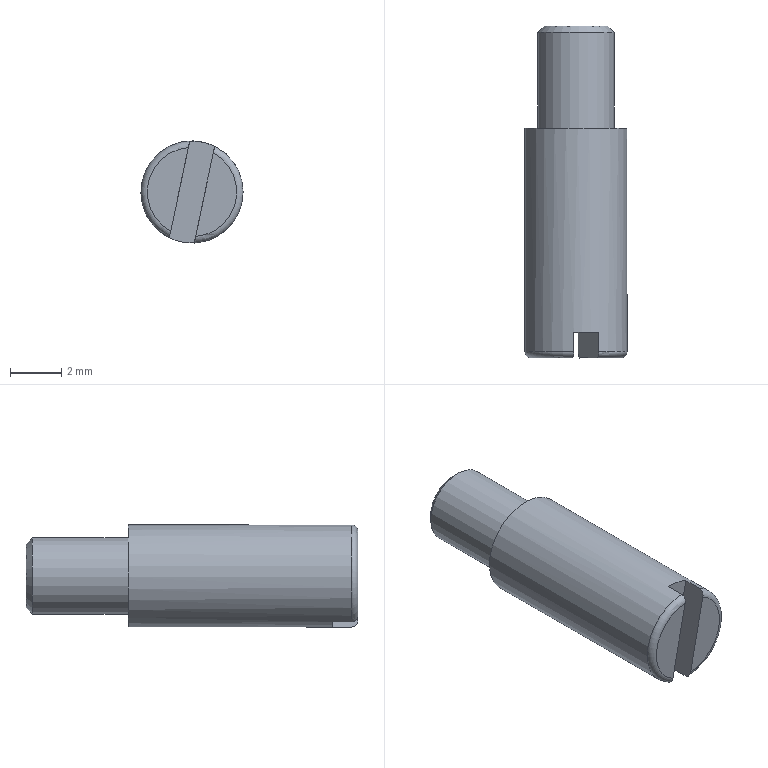Component | NX | PIN | 1 solid | 12 faces | volume 137 mm3 | plane 7 | cylinder 2 | torus 2 | cone 1 | commonest cylinder face diameters 4 x1 3 x1